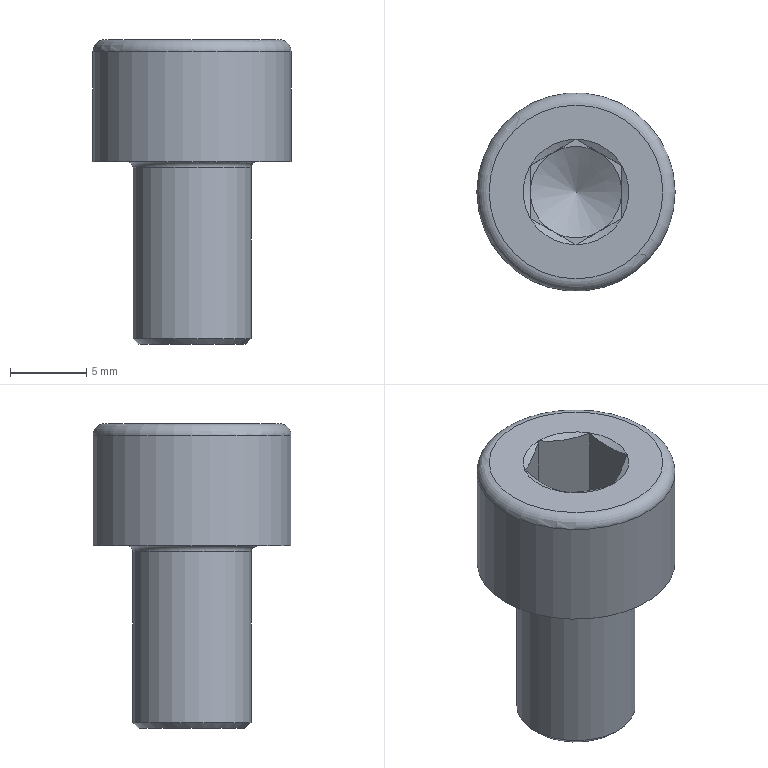Component | NX | GB-T70_1-2000_M8X12 | 1 solid | 27 faces | volume 1459 mm3 | plane 15 | cone 8 | cylinder 2 | torus 2 | commonest cylinder face diameters 7.76 x1 13 x1